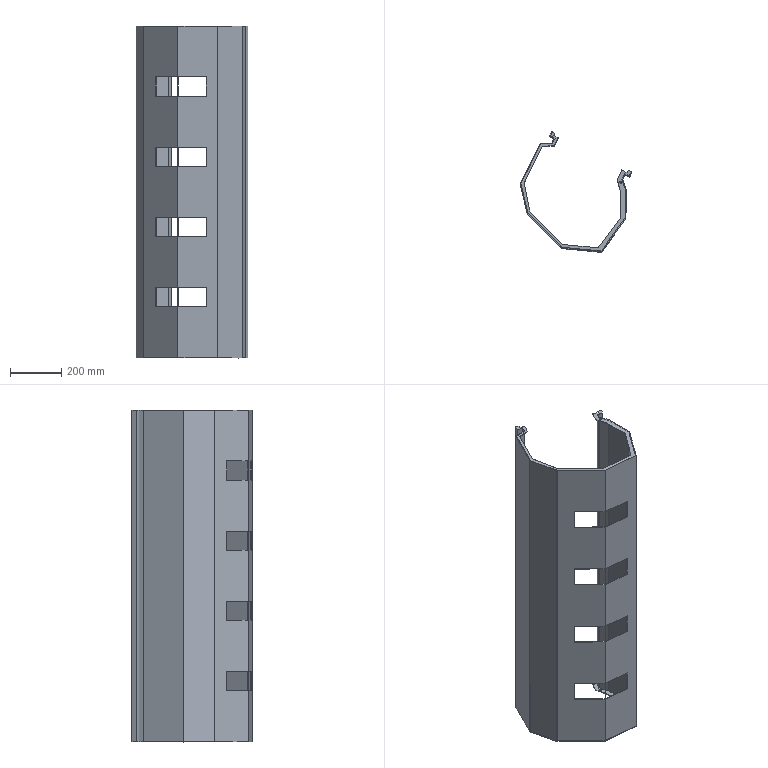Component | SolidWorks | SeedBoxAssemblyModified-1_SeedBoxModification-2 | 1 solid | 98 faces | volume 4178830 mm3 | plane 94 | cylinder 4 | commonest cylinder face diameters 9 x4